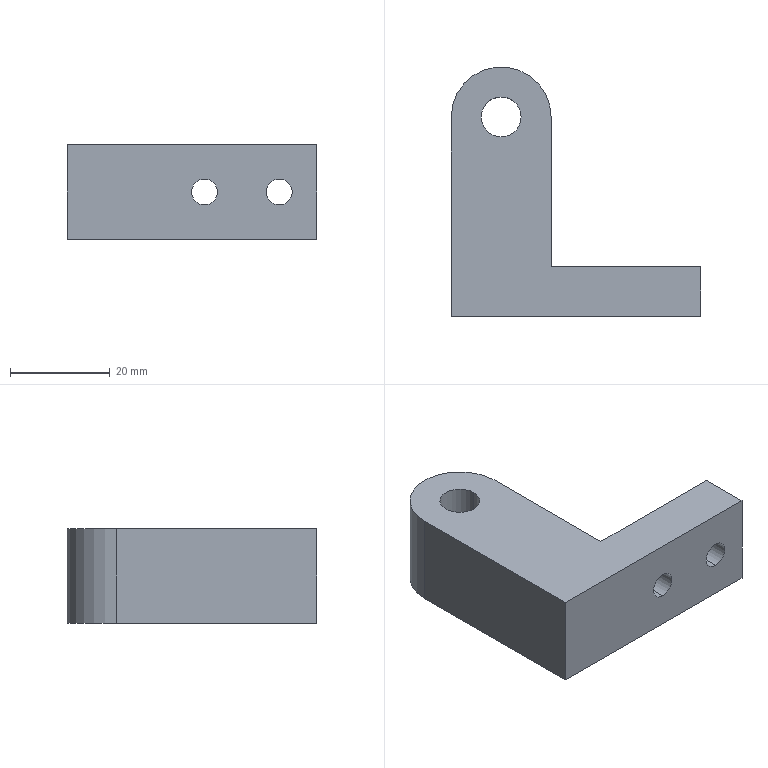Component | SolidWorks | TAR-02-022PaperPressWheelSeat-1 | 1 solid | 23 faces | box 50 x 50 x 19 mm | volume 21410 mm3 | cylinder 13 | plane 10 | commonest cylinder face diameters 9 x4 5.2 x4 12 x2 8 x2 20 x1
build123d program:
from build123d import *

# Parameters (mm, degrees)
SKETCH1_R                                            = 4
BOSS_EXTRUDE1_DEPTH                                  = 19
M5_HEX_HEAD_BOLT_CYLINDRICAL_COUNTERSUNK_D           = 5.2
M5_HEX_HEAD_BOLT_CYLINDRICAL_COUNTERSUNK_CBORE_D     = 9
M5_HEX_HEAD_BOLT_CYLINDRICAL_COUNTERSUNK_CBORE_DEPTH = 5.5
SKETCH5_R                                            = 6
CUT_EXTRUDE1_DEPTH                                   = 10


with BuildPart() as part:
    # Sketch1 → Boss-Extrude1 (new body)
    with BuildSketch(Plane.XY):
        with BuildLine():
            Line((-68.625, 16.452), (-68.625, -23.548))
            Line((-68.625, -23.548), (-18.625, -23.548))
            Line((-18.625, -23.548), (-18.625, -13.548))
            Line((-18.625, -13.548), (-48.625, -13.548))
            Line((-48.625, -13.548), (-48.625, -4.548))
            Line((-48.625, -4.548), (-48.625, -3.548))
            Line((-48.625, -3.548), (-48.625, 16.452))
            ThreePointArc((-48.625, 16.452), (-58.625, 26.452), (-68.625, 16.452))
        make_face()
        with Locations((-58.625, 16.452)):
            Circle(SKETCH1_R, mode=Mode.SUBTRACT)
    extrude(amount=BOSS_EXTRUDE1_DEPTH)

    # M5 Hex Head Bolt Cylindrical Countersunk (through all)
    with Locations(Plane(origin=(-41.125, -13.548, 9.5), x_dir=(1, 0, 0), z_dir=(0, 1, 0))):
        with Locations((0, 0), (15, 0)):
            CounterBoreHole(M5_HEX_HEAD_BOLT_CYLINDRICAL_COUNTERSUNK_D / 2, M5_HEX_HEAD_BOLT_CYLINDRICAL_COUNTERSUNK_CBORE_D / 2, M5_HEX_HEAD_BOLT_CYLINDRICAL_COUNTERSUNK_CBORE_DEPTH)

    # Sketch5 → Cut-Extrude1 (cut)
    with BuildSketch(Plane(origin=(0, 0, 0), x_dir=(-1, 0, 0), z_dir=(0, 0, -1))):
        with Locations((58.625, 16.452)):
            Circle(SKETCH5_R)
    extrude(amount=-CUT_EXTRUDE1_DEPTH, mode=Mode.SUBTRACT)


solid = part.part

# Placed as in the assembly
solid = solid.moved(Location((12.734, 52.336, -9.5), (0, 0, 0)))
STEP:
#1=CARTESIAN_POINT('',(-1.571,2.708,0.01969));
#2=VERTEX_POINT('',#1);
#3=CARTESIAN_POINT('',(-2.043,2.708,0.01969));
#4=VERTEX_POINT('',#3);
#5=CARTESIAN_POINT('',(-1.807,2.708,0.01969));
#6=DIRECTION('',(0.,0.,-1.));
#7=DIRECTION('',(-1.,0.,0.));
#8=AXIS2_PLACEMENT_3D('',#5,#6,#7);
#9=CIRCLE('',#8,0.2362);
#10=EDGE_CURVE('',#2,#4,#9,.T.);
#11=ORIENTED_EDGE('',*,*,#10,.F.);
#12=CARTESIAN_POINT('',(-1.571,2.708,-0.374));
#13=VERTEX_POINT('',#12);
#14=CARTESIAN_POINT('',(-1.571,2.708,0.01969));
#15=DIRECTION('',(0.,0.,-1.));
#16=VECTOR('',#15,39.37);
#17=LINE('',#14,#16);
#18=EDGE_CURVE('',#2,#13,#17,.T.);
#19=ORIENTED_EDGE('',*,*,#18,.T.);
#20=CARTESIAN_POINT('',(-2.043,2.708,-0.374));
#21=VERTEX_POINT('',#20);
#22=CARTESIAN_POINT('',(-1.807,2.708,-0.374));
#23=DIRECTION('',(0.,0.,-1.));
#24=DIRECTION('',(-1.,0.,0.));
#25=AXIS2_PLACEMENT_3D('',#22,#23,#24);
#26=CIRCLE('',#25,0.2362);
#27=EDGE_CURVE('',#13,#21,#26,.T.);
#28=ORIENTED_EDGE('',*,*,#27,.T.);
#29=CARTESIAN_POINT('',(-2.043,2.708,0.01969));
#30=DIRECTION('',(0.,0.,-1.));
#31=VECTOR('',#30,39.37);
#32=LINE('',#29,#31);
#33=EDGE_CURVE('',#4,#21,#32,.T.);
#34=ORIENTED_EDGE('',*,*,#33,.F.);
#35=EDGE_LOOP('',(#11,#19,#28,#34));
#36=FACE_OUTER_BOUND('',#35,.T.);
#37=CARTESIAN_POINT('',(-1.807,2.708,0.01969));
#38=DIRECTION('',(0.,0.,-1.));
#39=DIRECTION('',(-1.,0.,0.));
#40=AXIS2_PLACEMENT_3D('',#37,#38,#39);
#41=CYLINDRICAL_SURFACE('',#40,0.2362);
#42=ADVANCED_FACE('',(#36),#41,.F.);
#43=CARTESIAN_POINT('',(-1.118,1.311,-0.1772));
#44=VERTEX_POINT('',#43);
#45=CARTESIAN_POINT('',(-1.118,1.311,0.1772));
#46=VERTEX_POINT('',#45);
#47=CARTESIAN_POINT('',(-1.118,1.311,0.));
#48=DIRECTION('',(0.,1.,0.));
#49=DIRECTION('',(0.,0.,1.));
#50=AXIS2_PLACEMENT_3D('',#47,#48,#49);
#51=CIRCLE('',#50,0.1772);
#52=EDGE_CURVE('',#44,#46,#51,.T.);
#53=ORIENTED_EDGE('',*,*,#52,.F.);
#54=CARTESIAN_POINT('',(-1.118,1.527,-0.1772));
#55=VERTEX_POINT('',#54);
#56=CARTESIAN_POINT('',(-1.118,1.527,-0.1772));
#57=DIRECTION('',(0.,1.,0.));
#58=VECTOR('',#57,39.37);
#59=LINE('',#56,#58);
#60=EDGE_CURVE('',#44,#55,#59,.T.);
#61=ORIENTED_EDGE('',*,*,#60,.T.);
#62=CARTESIAN_POINT('',(-1.118,1.527,0.1772));
#63=VERTEX_POINT('',#62);
#64=CARTESIAN_POINT('',(-1.118,1.527,0.));
#65=DIRECTION('',(0.,1.,0.));
#66=DIRECTION('',(0.,0.,1.));
#67=AXIS2_PLACEMENT_3D('',#64,#65,#66);
#68=CIRCLE('',#67,0.1772);
#69=EDGE_CURVE('',#55,#63,#68,.T.);
#70=ORIENTED_EDGE('',*,*,#69,.T.);
#71=CARTESIAN_POINT('',(-1.118,1.527,0.1772));
#72=DIRECTION('',(0.,1.,0.));
#73=VECTOR('',#72,39.37);
#74=LINE('',#71,#73);
#75=EDGE_CURVE('',#46,#63,#74,.T.);
#76=ORIENTED_EDGE('',*,*,#75,.F.);
#77=EDGE_LOOP('',(#53,#61,#70,#76));
#78=FACE_OUTER_BOUND('',#77,.T.);
#79=CARTESIAN_POINT('',(-1.118,1.527,0.));
#80=DIRECTION('',(0.,1.,0.));
#81=DIRECTION('',(0.,0.,1.));
#82=AXIS2_PLACEMENT_3D('',#79,#80,#81);
#83=CYLINDRICAL_SURFACE('',#82,0.1772);
#84=ADVANCED_FACE('',(#78),#83,.F.);
#85=CARTESIAN_POINT('',(-1.118,1.133,-0.1024));
#86=VERTEX_POINT('',#85);
#87=CARTESIAN_POINT('',(-1.118,1.133,0.1024));
#88=VERTEX_POINT('',#87);
#89=CARTESIAN_POINT('',(-1.118,1.133,0.));
#90=DIRECTION('',(0.,1.,0.));
#91=DIRECTION('',(0.,0.,1.));
#92=AXIS2_PLACEMENT_3D('',#89,#90,#91);
#93=CIRCLE('',#92,0.1024);
#94=EDGE_CURVE('',#86,#88,#93,.T.);
#95=ORIENTED_EDGE('',*,*,#94,.F.);
#96=CARTESIAN_POINT('',(-1.118,1.311,-0.1024));
#97=VERTEX_POINT('',#96);
#98=CARTESIAN_POINT('',(-1.118,1.527,-0.1024));
#99=DIRECTION('',(0.,1.,0.));
#100=VECTOR('',#99,39.37);
#101=LINE('',#98,#100);
#102=EDGE_CURVE('',#86,#97,#101,.T.);
#103=ORIENTED_EDGE('',*,*,#102,.T.);
#104=CARTESIAN_POINT('',(-1.118,1.311,0.1024));
#105=VERTEX_POINT('',#104);
#106=CARTESIAN_POINT('',(-1.118,1.311,0.));
#107=DIRECTION('',(0.,1.,0.));
#108=DIRECTION('',(0.,0.,1.));
#109=AXIS2_PLACEMENT_3D('',#106,#107,#108);
#110=CIRCLE('',#109,0.1024);
#111=EDGE_CURVE('',#97,#105,#110,.T.);
#112=ORIENTED_EDGE('',*,*,#111,.T.);
#113=CARTESIAN_POINT('',(-1.118,1.527,0.1024));
#114=DIRECTION('',(0.,1.,0.));
#115=VECTOR('',#114,39.37);
#116=LINE('',#113,#115);
#117=EDGE_CURVE('',#88,#105,#116,.T.);
#118=ORIENTED_EDGE('',*,*,#117,.F.);
#119=EDGE_LOOP('',(#95,#103,#112,#118));
#120=FACE_OUTER_BOUND('',#119,.T.);
#121=CARTESIAN_POINT('',(-1.118,1.527,0.));
#122=DIRECTION('',(0.,1.,0.));
#123=DIRECTION('',(0.,0.,1.));
#124=AXIS2_PLACEMENT_3D('',#121,#122,#123);
#125=CYLINDRICAL_SURFACE('',#124,0.1024);
#126=ADVANCED_FACE('',(#120),#125,.F.);
#127=CARTESIAN_POINT('',(-0.5272,1.311,-0.1772));
#128=VERTEX_POINT('',#127);
#129=CARTESIAN_POINT('',(-0.5272,1.311,0.1772));
#130=VERTEX_POINT('',#129);
#131=CARTESIAN_POINT('',(-0.5272,1.311,0.));
#132=DIRECTION('',(0.,1.,0.));
#133=DIRECTION('',(0.,0.,1.));
#134=AXIS2_PLACEMENT_3D('',#131,#132,#133);
#135=CIRCLE('',#134,0.1772);
#136=EDGE_CURVE('',#128,#130,#135,.T.);
#137=ORIENTED_EDGE('',*,*,#136,.F.);
#138=CARTESIAN_POINT('',(-0.5272,1.527,-0.1772));
#139=VERTEX_POINT('',#138);
#140=CARTESIAN_POINT('',(-0.5272,1.527,-0.1772));
#141=DIRECTION('',(0.,1.,0.));
#142=VECTOR('',#141,39.37);
#143=LINE('',#140,#142);
#144=EDGE_CURVE('',#128,#139,#143,.T.);
#145=ORIENTED_EDGE('',*,*,#144,.T.);
#146=CARTESIAN_POINT('',(-0.5272,1.527,0.1772));
#147=VERTEX_POINT('',#146);
#148=CARTESIAN_POINT('',(-0.5272,1.527,0.));
#149=DIRECTION('',(0.,1.,0.));
#150=DIRECTION('',(0.,0.,1.));
#151=AXIS2_PLACEMENT_3D('',#148,#149,#150);
#152=CIRCLE('',#151,0.1772);
#153=EDGE_CURVE('',#139,#147,#152,.T.);
#154=ORIENTED_EDGE('',*,*,#153,.T.);
#155=CARTESIAN_POINT('',(-0.5272,1.527,0.1772));
#156=DIRECTION('',(0.,1.,0.));
#157=VECTOR('',#156,39.37);
#158=LINE('',#155,#157);
#159=EDGE_CURVE('',#130,#147,#158,.T.);
#160=ORIENTED_EDGE('',*,*,#159,.F.);
#161=EDGE_LOOP('',(#137,#145,#154,#160));
#162=FACE_OUTER_BOUND('',#161,.T.);
#163=CARTESIAN_POINT('',(-0.5272,1.527,0.));
#164=DIRECTION('',(0.,1.,0.));
#165=DIRECTION('',(0.,0.,1.));
#166=AXIS2_PLACEMENT_3D('',#163,#164,#165);
#167=CYLINDRICAL_SURFACE('',#166,0.1772);
#168=ADVANCED_FACE('',(#162),#167,.F.);
#169=CARTESIAN_POINT('',(-0.5272,1.133,-0.1024));
#170=VERTEX_POINT('',#169);
#171=CARTESIAN_POINT('',(-0.5272,1.133,0.1024));
#172=VERTEX_POINT('',#171);
#173=CARTESIAN_POINT('',(-0.5272,1.133,0.));
#174=DIRECTION('',(0.,1.,0.));
#175=DIRECTION('',(0.,0.,1.));
#176=AXIS2_PLACEMENT_3D('',#173,#174,#175);
#177=CIRCLE('',#176,0.1024);
#178=EDGE_CURVE('',#170,#172,#177,.T.);
#179=ORIENTED_EDGE('',*,*,#178,.F.);
#180=CARTESIAN_POINT('',(-0.5272,1.311,-0.1024));
#181=VERTEX_POINT('',#180);
#182=CARTESIAN_POINT('',(-0.5272,1.527,-0.1024));
#183=DIRECTION('',(0.,1.,0.));
#184=VECTOR('',#183,39.37);
#185=LINE('',#182,#184);
#186=EDGE_CURVE('',#170,#181,#185,.T.);
#187=ORIENTED_EDGE('',*,*,#186,.T.);
#188=CARTESIAN_POINT('',(-0.5272,1.311,0.1024));
#189=VERTEX_POINT('',#188);
#190=CARTESIAN_POINT('',(-0.5272,1.311,0.));
#191=DIRECTION('',(0.,1.,0.));
#192=DIRECTION('',(0.,0.,1.));
#193=AXIS2_PLACEMENT_3D('',#190,#191,#192);
#194=CIRCLE('',#193,0.1024);
#195=EDGE_CURVE('',#181,#189,#194,.T.);
#196=ORIENTED_EDGE('',*,*,#195,.T.);
#197=CARTESIAN_POINT('',(-0.5272,1.527,0.1024));
#198=DIRECTION('',(0.,1.,0.));
#199=VECTOR('',#198,39.37);
#200=LINE('',#197,#199);
#201=EDGE_CURVE('',#172,#189,#200,.T.);
#202=ORIENTED_EDGE('',*,*,#201,.F.);
#203=EDGE_LOOP('',(#179,#187,#196,#202));
#204=FACE_OUTER_BOUND('',#203,.T.);
#205=CARTESIAN_POINT('',(-0.5272,1.527,0.));
#206=DIRECTION('',(0.,1.,0.));
#207=DIRECTION('',(0.,0.,1.));
#208=AXIS2_PLACEMENT_3D('',#205,#206,#207);
#209=CYLINDRICAL_SURFACE('',#208,0.1024);
#210=ADVANCED_FACE('',(#204),#209,.F.);
#211=CARTESIAN_POINT('',(-1.964,2.708,0.374));
#212=VERTEX_POINT('',#211);
#213=CARTESIAN_POINT('',(-1.649,2.708,0.374));
#214=VERTEX_POINT('',#213);
#215=CARTESIAN_POINT('',(-1.807,2.708,0.374));
#216=DIRECTION('',(0.,0.,1.));
#217=DIRECTION('',(1.,0.,0.));
#218=AXIS2_PLACEMENT_3D('',#215,#216,#217);
#219=CIRCLE('',#218,0.1575);
#220=EDGE_CURVE('',#212,#214,#219,.T.);
#221=ORIENTED_EDGE('',*,*,#220,.T.);
#222=CARTESIAN_POINT('',(-1.649,2.708,0.01969));
#223=VERTEX_POINT('',#222);
#224=CARTESIAN_POINT('',(-1.649,2.708,0.374));
#225=DIRECTION('',(0.,0.,-1.));
#226=VECTOR('',#225,39.37);
#227=LINE('',#224,#226);
#228=EDGE_CURVE('',#214,#223,#227,.T.);
#229=ORIENTED_EDGE('',*,*,#228,.T.);
#230=CARTESIAN_POINT('',(-1.964,2.708,0.01969));
#231=VERTEX_POINT('',#230);
#232=CARTESIAN_POINT('',(-1.807,2.708,0.01969));
#233=DIRECTION('',(0.,0.,-1.));
#234=DIRECTION('',(-1.,0.,0.));
#235=AXIS2_PLACEMENT_3D('',#232,#233,#234);
#236=CIRCLE('',#235,0.1575);
#237=EDGE_CURVE('',#223,#231,#236,.T.);
#238=ORIENTED_EDGE('',*,*,#237,.T.);
#239=CARTESIAN_POINT('',(-1.964,2.708,0.374));
#240=DIRECTION('',(0.,0.,-1.));
#241=VECTOR('',#240,39.37);
#242=LINE('',#239,#241);
#243=EDGE_CURVE('',#212,#231,#242,.T.);
#244=ORIENTED_EDGE('',*,*,#243,.F.);
#245=EDGE_LOOP('',(#221,#229,#238,#244));
#246=FACE_OUTER_BOUND('',#245,.T.);
#247=CARTESIAN_POINT('',(-1.807,2.708,0.374));
#248=DIRECTION('',(0.,0.,-1.));
#249=DIRECTION('',(-1.,0.,0.));
#250=AXIS2_PLACEMENT_3D('',#247,#248,#249);
#251=CYLINDRICAL_SURFACE('',#250,0.1575);
#252=ADVANCED_FACE('',(#246),#251,.F.);
#253=ORIENTED_EDGE('',*,*,#228,.F.);
#254=CARTESIAN_POINT('',(-1.807,2.708,0.374));
#255=DIRECTION('',(0.,0.,1.));
#256=DIRECTION('',(1.,0.,0.));
#257=AXIS2_PLACEMENT_3D('',#254,#255,#256);
#258=CIRCLE('',#257,0.1575);
#259=EDGE_CURVE('',#214,#212,#258,.T.);
#260=ORIENTED_EDGE('',*,*,#259,.T.);
#261=ORIENTED_EDGE('',*,*,#243,.T.);
#262=CARTESIAN_POINT('',(-1.807,2.708,0.01969));
#263=DIRECTION('',(0.,0.,-1.));
#264=DIRECTION('',(-1.,0.,0.));
#265=AXIS2_PLACEMENT_3D('',#262,#263,#264);
#266=CIRCLE('',#265,0.1575);
#267=EDGE_CURVE('',#231,#223,#266,.T.);
#268=ORIENTED_EDGE('',*,*,#267,.T.);
#269=EDGE_LOOP('',(#253,#260,#261,#268));
#270=FACE_OUTER_BOUND('',#269,.T.);
#271=CARTESIAN_POINT('',(-1.807,2.708,0.374));
#272=DIRECTION('',(0.,0.,-1.));
#273=DIRECTION('',(-1.,0.,0.));
#274=AXIS2_PLACEMENT_3D('',#271,#272,#273);
#275=CYLINDRICAL_SURFACE('',#274,0.1575);
#276=ADVANCED_FACE('',(#270),#275,.F.);
#277=CARTESIAN_POINT('',(-1.413,2.708,0.374));
#278=VERTEX_POINT('',#277);
#279=CARTESIAN_POINT('',(-2.2,2.708,0.374));
#280=VERTEX_POINT('',#279);
#281=CARTESIAN_POINT('',(-1.807,2.708,0.374));
#282=DIRECTION('',(0.,0.,1.));
#283=DIRECTION('',(1.,0.,0.));
#284=AXIS2_PLACEMENT_3D('',#281,#282,#283);
#285=CIRCLE('',#284,0.3937);
#286=EDGE_CURVE('',#278,#280,#285,.T.);
#287=ORIENTED_EDGE('',*,*,#286,.T.);
#288=CARTESIAN_POINT('',(-2.2,1.133,0.374));
#289=VERTEX_POINT('',#288);
#290=CARTESIAN_POINT('',(-2.2,2.708,0.374));
#291=DIRECTION('',(0.,-1.,0.));
#292=VECTOR('',#291,39.37);
#293=LINE('',#290,#292);
#294=EDGE_CURVE('',#280,#289,#293,.T.);
#295=ORIENTED_EDGE('',*,*,#294,.T.);
#296=CARTESIAN_POINT('',(-0.2319,1.133,0.374));
#297=VERTEX_POINT('',#296);
#298=CARTESIAN_POINT('',(-2.2,1.133,0.374));
#299=DIRECTION('',(1.,0.,0.));
#300=VECTOR('',#299,39.37);
#301=LINE('',#298,#300);
#302=EDGE_CURVE('',#289,#297,#301,.T.);
#303=ORIENTED_EDGE('',*,*,#302,.T.);
#304=CARTESIAN_POINT('',(-0.2319,1.527,0.374));
#305=VERTEX_POINT('',#304);
#306=CARTESIAN_POINT('',(-0.2319,1.133,0.374));
#307=DIRECTION('',(0.,1.,0.));
#308=VECTOR('',#307,39.37);
#309=LINE('',#306,#308);
#310=EDGE_CURVE('',#297,#305,#309,.T.);
#311=ORIENTED_EDGE('',*,*,#310,.T.);
#312=CARTESIAN_POINT('',(-1.413,1.527,0.374));
#313=VERTEX_POINT('',#312);
#314=CARTESIAN_POINT('',(-0.2319,1.527,0.374));
#315=DIRECTION('',(-1.,-0.,0.));
#316=VECTOR('',#315,39.37);
#317=LINE('',#314,#316);
#318=EDGE_CURVE('',#305,#313,#317,.T.);
#319=ORIENTED_EDGE('',*,*,#318,.T.);
#320=CARTESIAN_POINT('',(-1.413,1.527,0.374));
#321=DIRECTION('',(0.,1.,0.));
#322=VECTOR('',#321,39.37);
#323=LINE('',#320,#322);
#324=EDGE_CURVE('',#313,#278,#323,.T.);
#325=ORIENTED_EDGE('',*,*,#324,.T.);
#326=EDGE_LOOP('',(#287,#295,#303,#311,#319,#325));
#327=FACE_OUTER_BOUND('',#326,.T.);
#328=ORIENTED_EDGE('',*,*,#220,.F.);
#329=ORIENTED_EDGE('',*,*,#259,.F.);
#330=EDGE_LOOP('',(#328,#329));
#331=FACE_BOUND('',#330,.T.);
#332=CARTESIAN_POINT('',(-1.807,2.708,0.374));
#333=DIRECTION('',(0.,0.,1.));
#334=DIRECTION('',(1.,0.,0.));
#335=AXIS2_PLACEMENT_3D('',#332,#333,#334);
#336=PLANE('',#335);
#337=ADVANCED_FACE('',(#327,#331),#336,.T.);
#338=CARTESIAN_POINT('',(-1.807,2.708,-0.374));
#339=DIRECTION('',(0.,0.,-1.));
#340=DIRECTION('',(-1.,0.,0.));
#341=AXIS2_PLACEMENT_3D('',#338,#339,#340);
#342=CIRCLE('',#341,0.2362);
#343=EDGE_CURVE('',#21,#13,#342,.T.);
#344=ORIENTED_EDGE('',*,*,#343,.F.);
#345=ORIENTED_EDGE('',*,*,#27,.F.);
#346=EDGE_LOOP('',(#344,#345));
#347=FACE_BOUND('',#346,.T.);
#348=CARTESIAN_POINT('',(-1.413,2.708,-0.374));
#349=VERTEX_POINT('',#348);
#350=CARTESIAN_POINT('',(-2.2,2.708,-0.374));
#351=VERTEX_POINT('',#350);
#352=CARTESIAN_POINT('',(-1.807,2.708,-0.374));
#353=DIRECTION('',(0.,0.,1.));
#354=DIRECTION('',(1.,0.,0.));
#355=AXIS2_PLACEMENT_3D('',#352,#353,#354);
#356=CIRCLE('',#355,0.3937);
#357=EDGE_CURVE('',#349,#351,#356,.T.);
#358=ORIENTED_EDGE('',*,*,#357,.F.);
#359=CARTESIAN_POINT('',(-1.413,1.527,-0.374));
#360=VERTEX_POINT('',#359);
#361=CARTESIAN_POINT('',(-1.413,1.921,-0.374));
#362=DIRECTION('',(-0.,1.,0.));
#363=VECTOR('',#362,39.37);
#364=LINE('',#361,#363);
#365=EDGE_CURVE('',#360,#349,#364,.T.);
#366=ORIENTED_EDGE('',*,*,#365,.F.);
#367=CARTESIAN_POINT('',(-0.2319,1.527,-0.374));
#368=VERTEX_POINT('',#367);
#369=CARTESIAN_POINT('',(-0.2319,1.527,-0.374));
#370=DIRECTION('',(-1.,-0.,0.));
#371=VECTOR('',#370,39.37);
#372=LINE('',#369,#371);
#373=EDGE_CURVE('',#368,#360,#372,.T.);
#374=ORIENTED_EDGE('',*,*,#373,.F.);
#375=CARTESIAN_POINT('',(-0.2319,1.133,-0.374));
#376=VERTEX_POINT('',#375);
#377=CARTESIAN_POINT('',(-0.2319,1.133,-0.374));
#378=DIRECTION('',(0.,1.,0.));
#379=VECTOR('',#378,39.37);
#380=LINE('',#377,#379);
#381=EDGE_CURVE('',#376,#368,#380,.T.);
#382=ORIENTED_EDGE('',*,*,#381,.F.);
#383=CARTESIAN_POINT('',(-2.2,1.133,-0.374));
#384=VERTEX_POINT('',#383);
#385=CARTESIAN_POINT('',(-2.2,1.133,-0.374));
#386=DIRECTION('',(1.,0.,0.));
#387=VECTOR('',#386,39.37);
#388=LINE('',#385,#387);
#389=EDGE_CURVE('',#384,#376,#388,.T.);
#390=ORIENTED_EDGE('',*,*,#389,.F.);
#391=CARTESIAN_POINT('',(-2.2,2.708,-0.374));
#392=DIRECTION('',(0.,-1.,0.));
#393=VECTOR('',#392,39.37);
#394=LINE('',#391,#393);
#395=EDGE_CURVE('',#351,#384,#394,.T.);
#396=ORIENTED_EDGE('',*,*,#395,.F.);
#397=EDGE_LOOP('',(#358,#366,#374,#382,#390,#396));
#398=FACE_OUTER_BOUND('',#397,.T.);
#399=CARTESIAN_POINT('',(-1.807,2.708,-0.374));
#400=DIRECTION('',(0.,0.,1.));
#401=DIRECTION('',(1.,0.,0.));
#402=AXIS2_PLACEMENT_3D('',#399,#400,#401);
#403=PLANE('',#402);
#404=ADVANCED_FACE('',(#347,#398),#403,.F.);
#405=ORIENTED_EDGE('',*,*,#357,.T.);
#406=CARTESIAN_POINT('',(-2.2,2.708,0.374));
#407=DIRECTION('',(0.,0.,-1.));
#408=VECTOR('',#407,39.37);
#409=LINE('',#406,#408);
#410=EDGE_CURVE('',#280,#351,#409,.T.);
#411=ORIENTED_EDGE('',*,*,#410,.F.);
#412=ORIENTED_EDGE('',*,*,#286,.F.);
#413=CARTESIAN_POINT('',(-1.413,2.708,0.374));
#414=DIRECTION('',(0.,0.,-1.));
#415=VECTOR('',#414,39.37);
#416=LINE('',#413,#415);
#417=EDGE_CURVE('',#278,#349,#416,.T.);
#418=ORIENTED_EDGE('',*,*,#417,.T.);
#419=EDGE_LOOP('',(#405,#411,#412,#418));
#420=FACE_OUTER_BOUND('',#419,.T.);
#421=CARTESIAN_POINT('',(-1.807,2.708,0.374));
#422=DIRECTION('',(0.,0.,-1.));
#423=DIRECTION('',(-1.,0.,0.));
#424=AXIS2_PLACEMENT_3D('',#421,#422,#423);
#425=CYLINDRICAL_SURFACE('',#424,0.3937);
#426=ADVANCED_FACE('',(#420),#425,.T.);
#427=ORIENTED_EDGE('',*,*,#395,.T.);
#428=CARTESIAN_POINT('',(-2.2,1.133,0.374));
#429=DIRECTION('',(0.,0.,-1.));
#430=VECTOR('',#429,39.37);
#431=LINE('',#428,#430);
#432=EDGE_CURVE('',#289,#384,#431,.T.);
#433=ORIENTED_EDGE('',*,*,#432,.F.);
#434=ORIENTED_EDGE('',*,*,#294,.F.);
#435=ORIENTED_EDGE('',*,*,#410,.T.);
#436=EDGE_LOOP('',(#427,#433,#434,#435));
#437=FACE_OUTER_BOUND('',#436,.T.);
#438=CARTESIAN_POINT('',(-2.2,2.708,0.374));
#439=DIRECTION('',(1.,0.,0.));
#440=DIRECTION('',(0.,0.,-1.));
#441=AXIS2_PLACEMENT_3D('',#438,#439,#440);
#442=PLANE('',#441);
#443=ADVANCED_FACE('',(#437),#442,.F.);
#444=CARTESIAN_POINT('',(-1.118,1.133,0.));
#445=DIRECTION('',(0.,1.,0.));
#446=DIRECTION('',(0.,0.,1.));
#447=AXIS2_PLACEMENT_3D('',#444,#445,#446);
#448=CIRCLE('',#447,0.1024);
#449=EDGE_CURVE('',#88,#86,#448,.T.);
#450=ORIENTED_EDGE('',*,*,#449,.T.);
#451=ORIENTED_EDGE('',*,*,#94,.T.);
#452=EDGE_LOOP('',(#450,#451));
#453=FACE_BOUND('',#452,.T.);
#454=CARTESIAN_POINT('',(-0.5272,1.133,0.));
#455=DIRECTION('',(0.,1.,0.));
#456=DIRECTION('',(0.,0.,1.));
#457=AXIS2_PLACEMENT_3D('',#454,#455,#456);
#458=CIRCLE('',#457,0.1024);
#459=EDGE_CURVE('',#172,#170,#458,.T.);
#460=ORIENTED_EDGE('',*,*,#459,.T.);
#461=ORIENTED_EDGE('',*,*,#178,.T.);
#462=EDGE_LOOP('',(#460,#461));
#463=FACE_BOUND('',#462,.T.);
#464=ORIENTED_EDGE('',*,*,#389,.T.);
#465=CARTESIAN_POINT('',(-0.2319,1.133,0.374));
#466=DIRECTION('',(0.,0.,-1.));
#467=VECTOR('',#466,39.37);
#468=LINE('',#465,#467);
#469=EDGE_CURVE('',#297,#376,#468,.T.);
#470=ORIENTED_EDGE('',*,*,#469,.F.);
#471=ORIENTED_EDGE('',*,*,#302,.F.);
#472=ORIENTED_EDGE('',*,*,#432,.T.);
#473=EDGE_LOOP('',(#464,#470,#471,#472));
#474=FACE_OUTER_BOUND('',#473,.T.);
#475=CARTESIAN_POINT('',(-2.2,1.133,0.374));
#476=DIRECTION('',(-0.,1.,0.));
#477=DIRECTION('',(-1.,-0.,0.));
#478=AXIS2_PLACEMENT_3D('',#475,#476,#477);
#479=PLANE('',#478);
#480=ADVANCED_FACE('',(#453,#463,#474),#479,.F.);
#481=ORIENTED_EDGE('',*,*,#381,.T.);
#482=CARTESIAN_POINT('',(-0.2319,1.527,0.374));
#483=DIRECTION('',(0.,0.,-1.));
#484=VECTOR('',#483,39.37);
#485=LINE('',#482,#484);
#486=EDGE_CURVE('',#305,#368,#485,.T.);
#487=ORIENTED_EDGE('',*,*,#486,.F.);
#488=ORIENTED_EDGE('',*,*,#310,.F.);
#489=ORIENTED_EDGE('',*,*,#469,.T.);
#490=EDGE_LOOP('',(#481,#487,#488,#489));
#491=FACE_OUTER_BOUND('',#490,.T.);
#492=CARTESIAN_POINT('',(-0.2319,1.133,0.374));
#493=DIRECTION('',(-1.,0.,0.));
#494=DIRECTION('',(-0.,-1.,0.));
#495=AXIS2_PLACEMENT_3D('',#492,#493,#494);
#496=PLANE('',#495);
#497=ADVANCED_FACE('',(#491),#496,.F.);
#498=CARTESIAN_POINT('',(-1.118,1.527,0.));
#499=DIRECTION('',(0.,1.,0.));
#500=DIRECTION('',(0.,0.,1.));
#501=AXIS2_PLACEMENT_3D('',#498,#499,#500);
#502=CIRCLE('',#501,0.1772);
#503=EDGE_CURVE('',#63,#55,#502,.T.);
#504=ORIENTED_EDGE('',*,*,#503,.F.);
#505=ORIENTED_EDGE('',*,*,#69,.F.);
#506=EDGE_LOOP('',(#504,#505));
#507=FACE_BOUND('',#506,.T.);
#508=CARTESIAN_POINT('',(-0.5272,1.527,0.));
#509=DIRECTION('',(0.,1.,0.));
#510=DIRECTION('',(0.,0.,1.));
#511=AXIS2_PLACEMENT_3D('',#508,#509,#510);
#512=CIRCLE('',#511,0.1772);
#513=EDGE_CURVE('',#147,#139,#512,.T.);
#514=ORIENTED_EDGE('',*,*,#513,.F.);
#515=ORIENTED_EDGE('',*,*,#153,.F.);
#516=EDGE_LOOP('',(#514,#515));
#517=FACE_BOUND('',#516,.T.);
#518=ORIENTED_EDGE('',*,*,#373,.T.);
#519=CARTESIAN_POINT('',(-1.413,1.527,0.374));
#520=DIRECTION('',(0.,0.,-1.));
#521=VECTOR('',#520,39.37);
#522=LINE('',#519,#521);
#523=EDGE_CURVE('',#313,#360,#522,.T.);
#524=ORIENTED_EDGE('',*,*,#523,.F.);
#525=ORIENTED_EDGE('',*,*,#318,.F.);
#526=ORIENTED_EDGE('',*,*,#486,.T.);
#527=EDGE_LOOP('',(#518,#524,#525,#526));
#528=FACE_OUTER_BOUND('',#527,.T.);
#529=CARTESIAN_POINT('',(-0.2319,1.527,0.374));
#530=DIRECTION('',(0.,-1.,0.));
#531=DIRECTION('',(1.,0.,0.));
#532=AXIS2_PLACEMENT_3D('',#529,#530,#531);
#533=PLANE('',#532);
#534=ADVANCED_FACE('',(#507,#517,#528),#533,.F.);
#535=ORIENTED_EDGE('',*,*,#365,.T.);
#536=ORIENTED_EDGE('',*,*,#417,.F.);
#537=ORIENTED_EDGE('',*,*,#324,.F.);
#538=ORIENTED_EDGE('',*,*,#523,.T.);
#539=EDGE_LOOP('',(#535,#536,#537,#538));
#540=FACE_OUTER_BOUND('',#539,.T.);
#541=CARTESIAN_POINT('',(-1.413,1.921,0.374));
#542=DIRECTION('',(-1.,-0.,0.));
#543=DIRECTION('',(0.,-1.,0.));
#544=AXIS2_PLACEMENT_3D('',#541,#542,#543);
#545=PLANE('',#544);
#546=ADVANCED_FACE('',(#540),#545,.F.);
#547=ORIENTED_EDGE('',*,*,#186,.F.);
#548=ORIENTED_EDGE('',*,*,#459,.F.);
#549=ORIENTED_EDGE('',*,*,#201,.T.);
#550=CARTESIAN_POINT('',(-0.5272,1.311,0.));
#551=DIRECTION('',(0.,1.,0.));
#552=DIRECTION('',(0.,0.,1.));
#553=AXIS2_PLACEMENT_3D('',#550,#551,#552);
#554=CIRCLE('',#553,0.1024);
#555=EDGE_CURVE('',#189,#181,#554,.T.);
#556=ORIENTED_EDGE('',*,*,#555,.T.);
#557=EDGE_LOOP('',(#547,#548,#549,#556));
#558=FACE_OUTER_BOUND('',#557,.T.);
#559=CARTESIAN_POINT('',(-0.5272,1.527,0.));
#560=DIRECTION('',(0.,1.,0.));
#561=DIRECTION('',(0.,0.,1.));
#562=AXIS2_PLACEMENT_3D('',#559,#560,#561);
#563=CYLINDRICAL_SURFACE('',#562,0.1024);
#564=ADVANCED_FACE('',(#558),#563,.F.);
#565=ORIENTED_EDGE('',*,*,#555,.F.);
#566=ORIENTED_EDGE('',*,*,#195,.F.);
#567=EDGE_LOOP('',(#565,#566));
#568=FACE_BOUND('',#567,.T.);
#569=CARTESIAN_POINT('',(-0.5272,1.311,0.));
#570=DIRECTION('',(0.,1.,0.));
#571=DIRECTION('',(0.,0.,1.));
#572=AXIS2_PLACEMENT_3D('',#569,#570,#571);
#573=CIRCLE('',#572,0.1772);
#574=EDGE_CURVE('',#130,#128,#573,.T.);
#575=ORIENTED_EDGE('',*,*,#574,.T.);
#576=ORIENTED_EDGE('',*,*,#136,.T.);
#577=EDGE_LOOP('',(#575,#576));
#578=FACE_OUTER_BOUND('',#577,.T.);
#579=CARTESIAN_POINT('',(-0.4248,1.311,0.));
#580=DIRECTION('',(0.,-1.,0.));
#581=DIRECTION('',(0.,0.,-1.));
#582=AXIS2_PLACEMENT_3D('',#579,#580,#581);
#583=PLANE('',#582);
#584=ADVANCED_FACE('',(#568,#578),#583,.F.);
#585=ORIENTED_EDGE('',*,*,#144,.F.);
#586=ORIENTED_EDGE('',*,*,#574,.F.);
#587=ORIENTED_EDGE('',*,*,#159,.T.);
#588=ORIENTED_EDGE('',*,*,#513,.T.);
#589=EDGE_LOOP('',(#585,#586,#587,#588));
#590=FACE_OUTER_BOUND('',#589,.T.);
#591=CARTESIAN_POINT('',(-0.5272,1.527,0.));
#592=DIRECTION('',(0.,1.,0.));
#593=DIRECTION('',(0.,0.,1.));
#594=AXIS2_PLACEMENT_3D('',#591,#592,#593);
#595=CYLINDRICAL_SURFACE('',#594,0.1772);
#596=ADVANCED_FACE('',(#590),#595,.F.);
#597=ORIENTED_EDGE('',*,*,#102,.F.);
#598=ORIENTED_EDGE('',*,*,#449,.F.);
#599=ORIENTED_EDGE('',*,*,#117,.T.);
#600=CARTESIAN_POINT('',(-1.118,1.311,0.));
#601=DIRECTION('',(0.,1.,0.));
#602=DIRECTION('',(0.,0.,1.));
#603=AXIS2_PLACEMENT_3D('',#600,#601,#602);
#604=CIRCLE('',#603,0.1024);
#605=EDGE_CURVE('',#105,#97,#604,.T.);
#606=ORIENTED_EDGE('',*,*,#605,.T.);
#607=EDGE_LOOP('',(#597,#598,#599,#606));
#608=FACE_OUTER_BOUND('',#607,.T.);
#609=CARTESIAN_POINT('',(-1.118,1.527,0.));
#610=DIRECTION('',(0.,1.,0.));
#611=DIRECTION('',(0.,0.,1.));
#612=AXIS2_PLACEMENT_3D('',#609,#610,#611);
#613=CYLINDRICAL_SURFACE('',#612,0.1024);
#614=ADVANCED_FACE('',(#608),#613,.F.);
#615=ORIENTED_EDGE('',*,*,#605,.F.);
#616=ORIENTED_EDGE('',*,*,#111,.F.);
#617=EDGE_LOOP('',(#615,#616));
#618=FACE_BOUND('',#617,.T.);
#619=CARTESIAN_POINT('',(-1.118,1.311,0.));
#620=DIRECTION('',(0.,1.,0.));
#621=DIRECTION('',(0.,0.,1.));
#622=AXIS2_PLACEMENT_3D('',#619,#620,#621);
#623=CIRCLE('',#622,0.1772);
#624=EDGE_CURVE('',#46,#44,#623,.T.);
#625=ORIENTED_EDGE('',*,*,#624,.T.);
#626=ORIENTED_EDGE('',*,*,#52,.T.);
#627=EDGE_LOOP('',(#625,#626));
#628=FACE_OUTER_BOUND('',#627,.T.);
#629=CARTESIAN_POINT('',(-1.015,1.311,0.));
#630=DIRECTION('',(0.,-1.,0.));
#631=DIRECTION('',(0.,0.,-1.));
#632=AXIS2_PLACEMENT_3D('',#629,#630,#631);
#633=PLANE('',#632);
#634=ADVANCED_FACE('',(#618,#628),#633,.F.);
#635=ORIENTED_EDGE('',*,*,#60,.F.);
#636=ORIENTED_EDGE('',*,*,#624,.F.);
#637=ORIENTED_EDGE('',*,*,#75,.T.);
#638=ORIENTED_EDGE('',*,*,#503,.T.);
#639=EDGE_LOOP('',(#635,#636,#637,#638));
#640=FACE_OUTER_BOUND('',#639,.T.);
#641=CARTESIAN_POINT('',(-1.118,1.527,0.));
#642=DIRECTION('',(0.,1.,0.));
#643=DIRECTION('',(0.,0.,1.));
#644=AXIS2_PLACEMENT_3D('',#641,#642,#643);
#645=CYLINDRICAL_SURFACE('',#644,0.1772);
#646=ADVANCED_FACE('',(#640),#645,.F.);
#647=ORIENTED_EDGE('',*,*,#18,.F.);
#648=CARTESIAN_POINT('',(-1.807,2.708,0.01969));
#649=DIRECTION('',(0.,0.,-1.));
#650=DIRECTION('',(-1.,0.,0.));
#651=AXIS2_PLACEMENT_3D('',#648,#649,#650);
#652=CIRCLE('',#651,0.2362);
#653=EDGE_CURVE('',#4,#2,#652,.T.);
#654=ORIENTED_EDGE('',*,*,#653,.F.);
#655=ORIENTED_EDGE('',*,*,#33,.T.);
#656=ORIENTED_EDGE('',*,*,#343,.T.);
#657=EDGE_LOOP('',(#647,#654,#655,#656));
#658=FACE_OUTER_BOUND('',#657,.T.);
#659=CARTESIAN_POINT('',(-1.807,2.708,0.01969));
#660=DIRECTION('',(0.,0.,-1.));
#661=DIRECTION('',(-1.,0.,0.));
#662=AXIS2_PLACEMENT_3D('',#659,#660,#661);
#663=CYLINDRICAL_SURFACE('',#662,0.2362);
#664=ADVANCED_FACE('',(#658),#663,.F.);
#665=ORIENTED_EDGE('',*,*,#267,.F.);
#666=ORIENTED_EDGE('',*,*,#237,.F.);
#667=EDGE_LOOP('',(#665,#666));
#668=FACE_BOUND('',#667,.T.);
#669=ORIENTED_EDGE('',*,*,#653,.T.);
#670=ORIENTED_EDGE('',*,*,#10,.T.);
#671=EDGE_LOOP('',(#669,#670));
#672=FACE_OUTER_BOUND('',#671,.T.);
#673=CARTESIAN_POINT('',(-1.807,2.708,0.01969));
#674=DIRECTION('',(0.,0.,-1.));
#675=DIRECTION('',(-1.,0.,0.));
#676=AXIS2_PLACEMENT_3D('',#673,#674,#675);
#677=PLANE('',#676);
#678=ADVANCED_FACE('',(#668,#672),#677,.T.);
#679=CLOSED_SHELL('',(#42,#84,#126,#168,#210,#252,#276,#337,#404,#426,#443,#480,#497,#534,#546,#564,#584,#596,#614,#634,#646,#664,#678));
#680=MANIFOLD_SOLID_BREP('',#679);
#681=CARTESIAN_POINT('',(0.,0.,0.));
#682=DIRECTION('',(0.,0.,1.));
#683=DIRECTION('',(1.,0.,0.));
#684=AXIS2_PLACEMENT_3D('',#681,#682,#683);
#685=(LENGTH_UNIT()NAMED_UNIT(*)SI_UNIT($,.METRE.));
#686=LENGTH_MEASURE_WITH_UNIT(LENGTH_MEASURE(0.0254),#685);
#687=DIMENSIONAL_EXPONENTS(1.,0.,0.,0.,0.,0.,0.);
#688=(CONVERSION_BASED_UNIT('',#686)LENGTH_UNIT()NAMED_UNIT(#687));
#689=UNCERTAINTY_MEASURE_WITH_UNIT(LENGTH_MEASURE(0.00001),#688,'','');
#690=(NAMED_UNIT(*)PLANE_ANGLE_UNIT()SI_UNIT($,.RADIAN.));
#691=(NAMED_UNIT(*)SI_UNIT($,.STERADIAN.)SOLID_ANGLE_UNIT());
#692=(GEOMETRIC_REPRESENTATION_CONTEXT(3)GLOBAL_UNCERTAINTY_ASSIGNED_CONTEXT((#689))GLOBAL_UNIT_ASSIGNED_CONTEXT((#688,#690,#691))REPRESENTATION_CONTEXT('',''));
#693=ADVANCED_BREP_SHAPE_REPRESENTATION('',(#680,#684),#692);
#694=COLOUR_RGB('',0.7922,0.8196,0.9333);
#695=FILL_AREA_STYLE_COLOUR('',#694);
#696=FILL_AREA_STYLE('',(#695));
#697=SURFACE_STYLE_FILL_AREA(#696);
#698=SURFACE_SIDE_STYLE('',(#697));
#699=SURFACE_STYLE_USAGE(.BOTH.,#698);
#700=PRESENTATION_STYLE_ASSIGNMENT((#699));
#701=STYLED_ITEM('',(#700),#680);
#702=PRESENTATION_LAYER_ASSIGNMENT('','',(#701));
#703=(LENGTH_UNIT()NAMED_UNIT(*)SI_UNIT($,.METRE.));
#704=LENGTH_MEASURE_WITH_UNIT(LENGTH_MEASURE(0.0254),#703);
#705=DIMENSIONAL_EXPONENTS(1.,0.,0.,0.,0.,0.,0.);
#706=(CONVERSION_BASED_UNIT('',#704)LENGTH_UNIT()NAMED_UNIT(#705));
#707=UNCERTAINTY_MEASURE_WITH_UNIT(LENGTH_MEASURE(0.00001),#706,'','');
#708=(NAMED_UNIT(*)PLANE_ANGLE_UNIT()SI_UNIT($,.RADIAN.));
#709=(NAMED_UNIT(*)SI_UNIT($,.STERADIAN.)SOLID_ANGLE_UNIT());
#710=(GEOMETRIC_REPRESENTATION_CONTEXT(3)GLOBAL_UNCERTAINTY_ASSIGNED_CONTEXT((#707))GLOBAL_UNIT_ASSIGNED_CONTEXT((#706,#708,#709))REPRESENTATION_CONTEXT('',''));
#711=MECHANICAL_DESIGN_GEOMETRIC_PRESENTATION_REPRESENTATION('',(#701),#710);